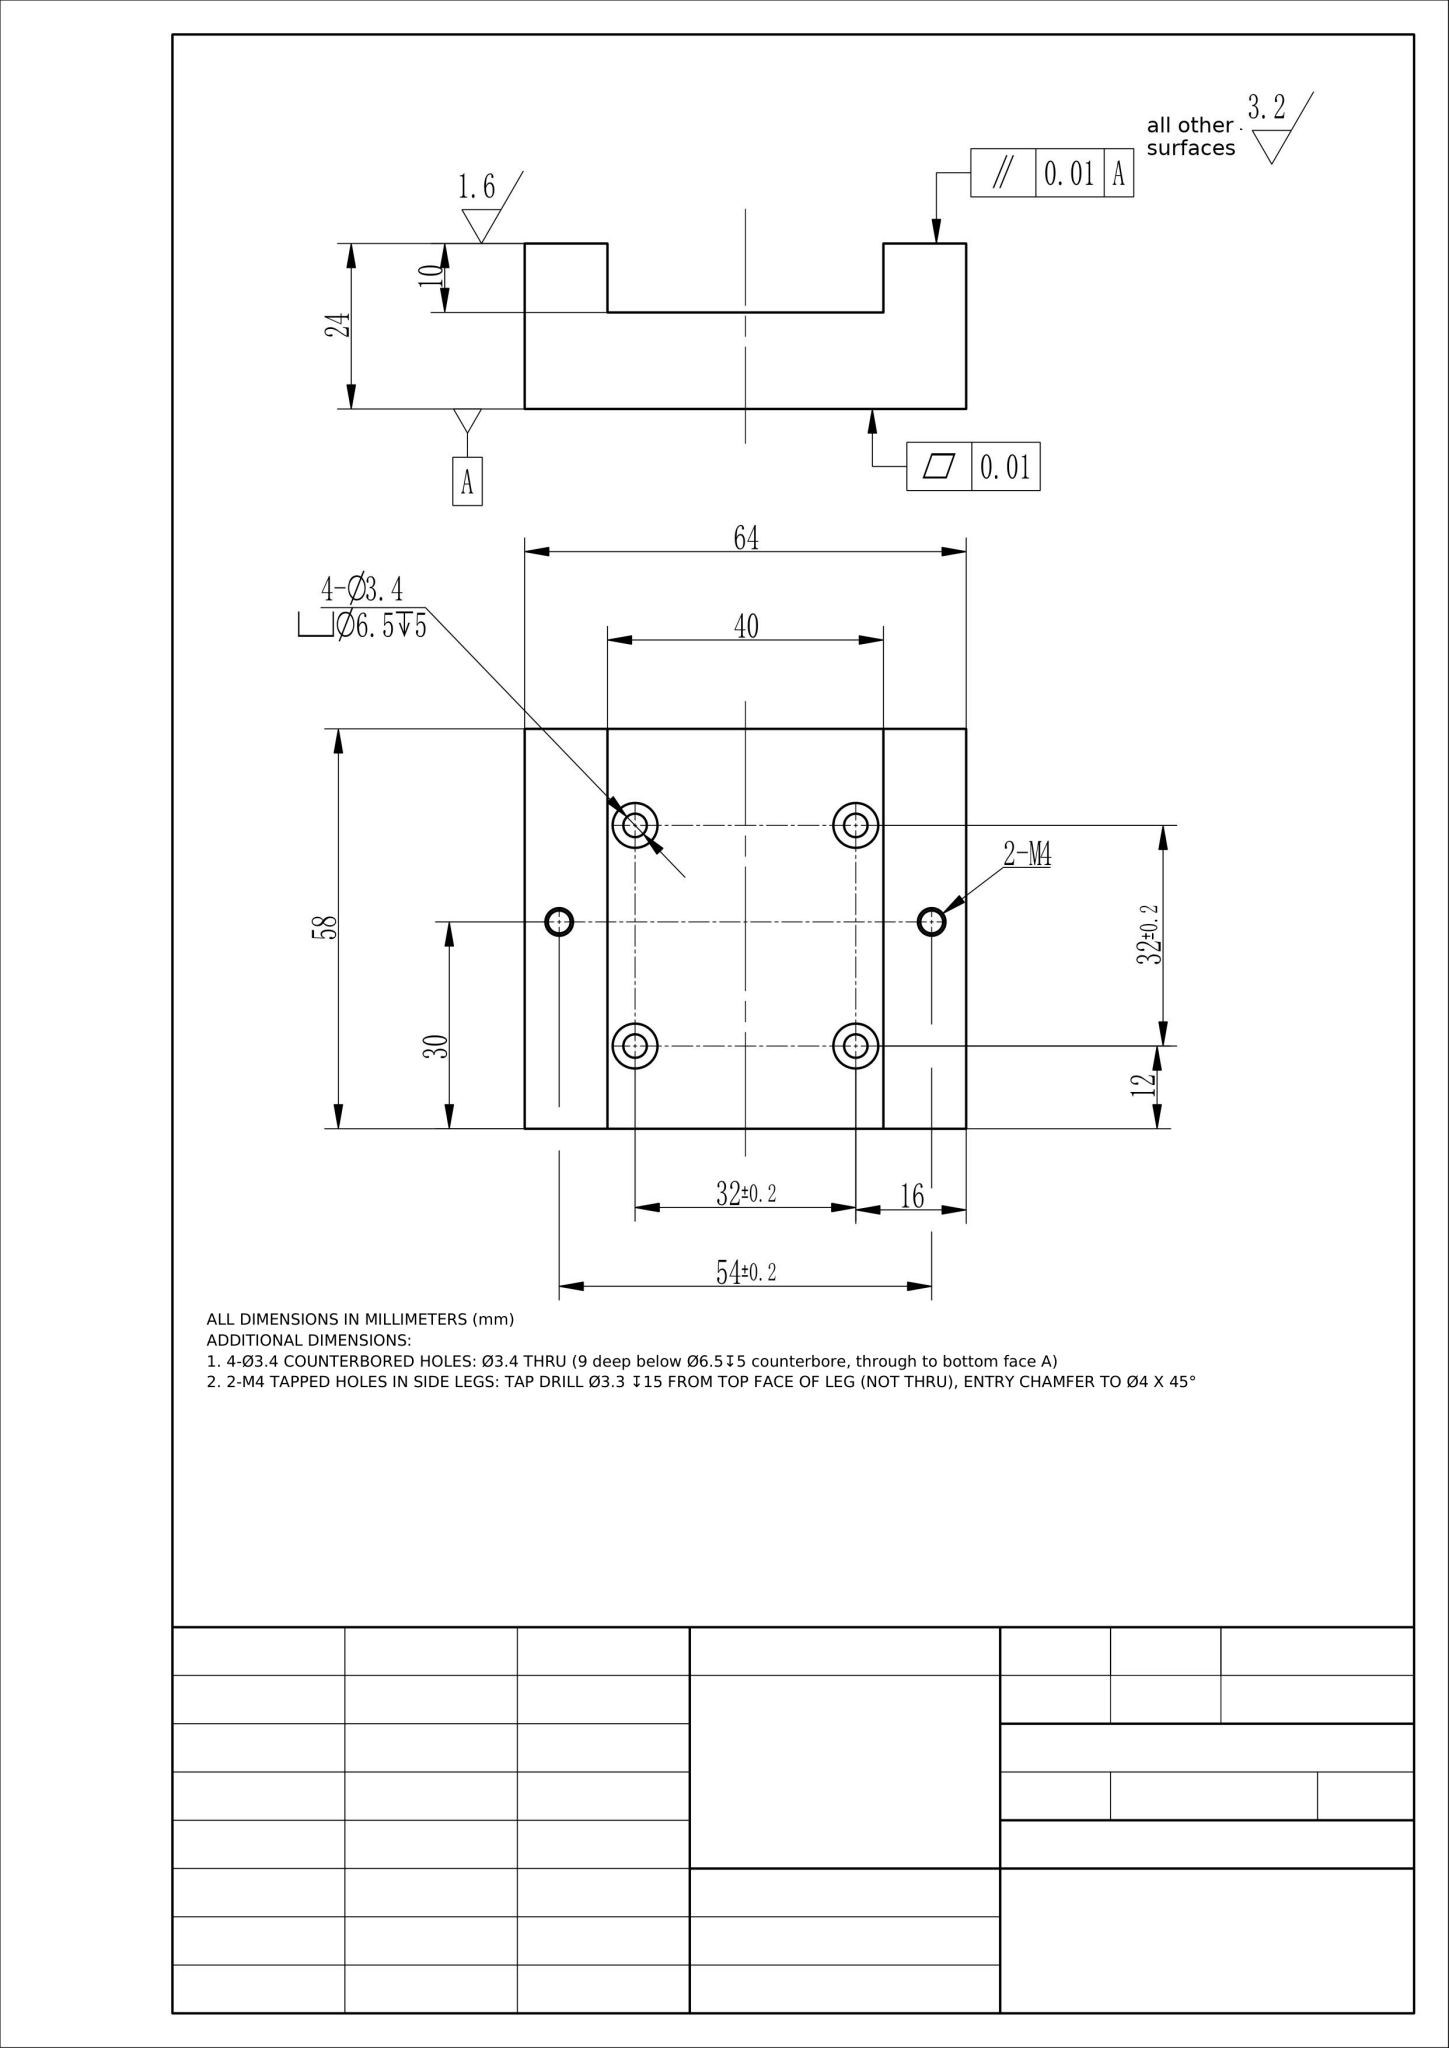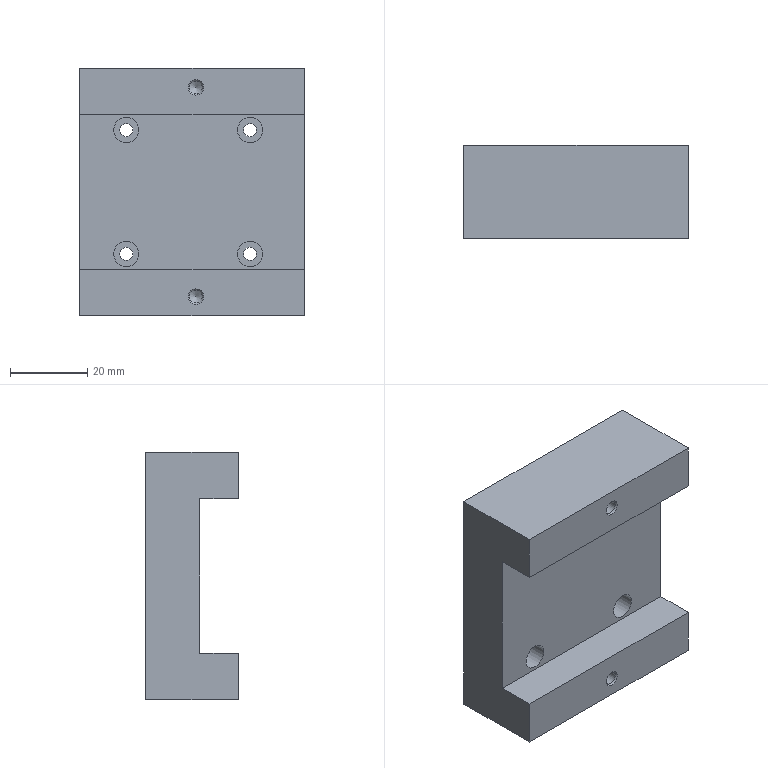Part | NX | mm | 1 solid | 28 faces | box 58 x 24 x 64 mm | volume 64634 mm3 | plane 14 | cylinder 10 | cone 4 | commonest cylinder face diameters 3.4 x4 6.5 x4 3.3 x2
STEP:
#1=CARTESIAN_POINT('',(0.,0.,0.));
#2=DIRECTION('',(0.,0.,1.));
#3=DIRECTION('',(1.,0.,0.));
#4=AXIS2_PLACEMENT_3D('',#1,#2,#3);
#5=(LENGTH_UNIT()NAMED_UNIT(*)SI_UNIT(.MILLI.,.METRE.));
#6=UNCERTAINTY_MEASURE_WITH_UNIT(LENGTH_MEASURE(0.00002),#5,'','');
#7=(NAMED_UNIT(*)PLANE_ANGLE_UNIT()SI_UNIT($,.RADIAN.));
#8=PLANE_ANGLE_MEASURE_WITH_UNIT(PLANE_ANGLE_MEASURE(0.01745),#7);
#9=DIMENSIONAL_EXPONENTS(0.,0.,0.,0.,0.,0.,0.);
#10=(CONVERSION_BASED_UNIT('',#8)NAMED_UNIT(#9)PLANE_ANGLE_UNIT());
#11=(NAMED_UNIT(*)SI_UNIT($,.STERADIAN.)SOLID_ANGLE_UNIT());
#12=(GEOMETRIC_REPRESENTATION_CONTEXT(3)GLOBAL_UNCERTAINTY_ASSIGNED_CONTEXT((#6))GLOBAL_UNIT_ASSIGNED_CONTEXT((#5,#10,#11))REPRESENTATION_CONTEXT('',''));
#13=SHAPE_REPRESENTATION('',(#4),#12);
#14=CARTESIAN_POINT('',(-56.,45.,156.029));
#15=VERTEX_POINT('',#14);
#16=CARTESIAN_POINT('',(-56.,55.,156.029));
#17=VERTEX_POINT('',#16);
#18=CARTESIAN_POINT('',(-56.,43.,156.029));
#19=DIRECTION('',(0.,1.,0.));
#20=VECTOR('',#19,1.);
#21=LINE('',#18,#20);
#22=EDGE_CURVE('',#15,#17,#21,.T.);
#23=ORIENTED_EDGE('',*,*,#22,.F.);
#24=CARTESIAN_POINT('',(-56.,45.,144.029));
#25=VERTEX_POINT('',#24);
#26=CARTESIAN_POINT('',(-56.,45.,154.029));
#27=DIRECTION('',(-0.,0.,1.));
#28=VECTOR('',#27,1.);
#29=LINE('',#26,#28);
#30=EDGE_CURVE('',#25,#15,#29,.T.);
#31=ORIENTED_EDGE('',*,*,#30,.F.);
#32=CARTESIAN_POINT('',(-56.,69.,144.029));
#33=VERTEX_POINT('',#32);
#34=CARTESIAN_POINT('',(-56.,45.,144.029));
#35=DIRECTION('',(0.,1.,0.));
#36=VECTOR('',#35,1.);
#37=LINE('',#34,#36);
#38=EDGE_CURVE('',#25,#33,#37,.T.);
#39=ORIENTED_EDGE('',*,*,#38,.T.);
#40=CARTESIAN_POINT('',(-56.,69.,208.029));
#41=VERTEX_POINT('',#40);
#42=CARTESIAN_POINT('',(-56.,69.,154.029));
#43=DIRECTION('',(-0.,0.,1.));
#44=VECTOR('',#43,1.);
#45=LINE('',#42,#44);
#46=EDGE_CURVE('',#33,#41,#45,.T.);
#47=ORIENTED_EDGE('',*,*,#46,.T.);
#48=CARTESIAN_POINT('',(-56.,45.,208.029));
#49=VERTEX_POINT('',#48);
#50=CARTESIAN_POINT('',(-56.,45.,208.029));
#51=DIRECTION('',(0.,1.,0.));
#52=VECTOR('',#51,1.);
#53=LINE('',#50,#52);
#54=EDGE_CURVE('',#49,#41,#53,.T.);
#55=ORIENTED_EDGE('',*,*,#54,.F.);
#56=CARTESIAN_POINT('',(-56.,45.,196.029));
#57=VERTEX_POINT('',#56);
#58=CARTESIAN_POINT('',(-56.,45.,154.029));
#59=DIRECTION('',(-0.,0.,1.));
#60=VECTOR('',#59,1.);
#61=LINE('',#58,#60);
#62=EDGE_CURVE('',#57,#49,#61,.T.);
#63=ORIENTED_EDGE('',*,*,#62,.F.);
#64=CARTESIAN_POINT('',(-56.,55.,196.029));
#65=VERTEX_POINT('',#64);
#66=CARTESIAN_POINT('',(-56.,55.,196.029));
#67=DIRECTION('',(0.,-1.,0.));
#68=VECTOR('',#67,1.);
#69=LINE('',#66,#68);
#70=EDGE_CURVE('',#65,#57,#69,.T.);
#71=ORIENTED_EDGE('',*,*,#70,.F.);
#72=CARTESIAN_POINT('',(-56.,55.,156.029));
#73=DIRECTION('',(0.,-0.,1.));
#74=VECTOR('',#73,1.);
#75=LINE('',#72,#74);
#76=EDGE_CURVE('',#17,#65,#75,.T.);
#77=ORIENTED_EDGE('',*,*,#76,.F.);
#78=EDGE_LOOP('',(#23,#31,#39,#47,#55,#63,#71,#77));
#79=FACE_OUTER_BOUND('',#78,.T.);
#80=CARTESIAN_POINT('',(-56.,45.,154.029));
#81=DIRECTION('',(-1.,0.,-0.));
#82=DIRECTION('',(-0.,0.,1.));
#83=AXIS2_PLACEMENT_3D('',#80,#81,#82);
#84=PLANE('',#83);
#85=ADVANCED_FACE('',(#79),#84,.F.);
#86=CARTESIAN_POINT('',(-114.,45.,156.029));
#87=VERTEX_POINT('',#86);
#88=CARTESIAN_POINT('',(0.,45.,156.029));
#89=DIRECTION('',(1.,0.,0.));
#90=VECTOR('',#89,1.);
#91=LINE('',#88,#90);
#92=EDGE_CURVE('',#87,#15,#91,.T.);
#93=ORIENTED_EDGE('',*,*,#92,.F.);
#94=CARTESIAN_POINT('',(-114.,45.,144.029));
#95=VERTEX_POINT('',#94);
#96=CARTESIAN_POINT('',(-114.,45.,198.029));
#97=DIRECTION('',(0.,0.,-1.));
#98=VECTOR('',#97,1.);
#99=LINE('',#96,#98);
#100=EDGE_CURVE('',#87,#95,#99,.T.);
#101=ORIENTED_EDGE('',*,*,#100,.T.);
#102=CARTESIAN_POINT('',(-111.,45.,144.029));
#103=DIRECTION('',(1.,0.,0.));
#104=VECTOR('',#103,1.);
#105=LINE('',#102,#104);
#106=EDGE_CURVE('',#95,#25,#105,.T.);
#107=ORIENTED_EDGE('',*,*,#106,.T.);
#108=ORIENTED_EDGE('',*,*,#30,.T.);
#109=EDGE_LOOP('',(#93,#101,#107,#108));
#110=FACE_BOUND('',#109,.T.);
#111=CARTESIAN_POINT('',(-84.,45.,147.029));
#112=VERTEX_POINT('',#111);
#113=CARTESIAN_POINT('',(-84.,45.,149.029));
#114=DIRECTION('',(0.,1.,0.));
#115=DIRECTION('',(0.,0.,-1.));
#116=AXIS2_PLACEMENT_3D('',#113,#114,#115);
#117=CIRCLE('',#116,2.);
#118=EDGE_CURVE('',#112,#112,#117,.T.);
#119=ORIENTED_EDGE('',*,*,#118,.T.);
#120=EDGE_LOOP('',(#119));
#121=FACE_BOUND('',#120,.T.);
#122=CARTESIAN_POINT('',(0.,45.,0.));
#123=DIRECTION('',(0.,-1.,0.));
#124=DIRECTION('',(0.,0.,-1.));
#125=AXIS2_PLACEMENT_3D('',#122,#123,#124);
#126=PLANE('',#125);
#127=ADVANCED_FACE('',(#110,#121),#126,.T.);
#128=ORIENTED_EDGE('',*,*,#100,.F.);
#129=CARTESIAN_POINT('',(-114.,55.,156.029));
#130=VERTEX_POINT('',#129);
#131=CARTESIAN_POINT('',(-114.,45.,156.029));
#132=DIRECTION('',(0.,1.,0.));
#133=VECTOR('',#132,1.);
#134=LINE('',#131,#133);
#135=EDGE_CURVE('',#87,#130,#134,.T.);
#136=ORIENTED_EDGE('',*,*,#135,.T.);
#137=CARTESIAN_POINT('',(-114.,55.,196.029));
#138=VERTEX_POINT('',#137);
#139=CARTESIAN_POINT('',(-114.,55.,198.029));
#140=DIRECTION('',(-0.,-0.,1.));
#141=VECTOR('',#140,1.);
#142=LINE('',#139,#141);
#143=EDGE_CURVE('',#130,#138,#142,.T.);
#144=ORIENTED_EDGE('',*,*,#143,.T.);
#145=CARTESIAN_POINT('',(-114.,45.,196.029));
#146=VERTEX_POINT('',#145);
#147=CARTESIAN_POINT('',(-114.,45.,196.029));
#148=DIRECTION('',(0.,-1.,0.));
#149=VECTOR('',#148,1.);
#150=LINE('',#147,#149);
#151=EDGE_CURVE('',#138,#146,#150,.T.);
#152=ORIENTED_EDGE('',*,*,#151,.T.);
#153=CARTESIAN_POINT('',(-114.,45.,208.029));
#154=VERTEX_POINT('',#153);
#155=CARTESIAN_POINT('',(-114.,45.,198.029));
#156=DIRECTION('',(0.,0.,-1.));
#157=VECTOR('',#156,1.);
#158=LINE('',#155,#157);
#159=EDGE_CURVE('',#154,#146,#158,.T.);
#160=ORIENTED_EDGE('',*,*,#159,.F.);
#161=CARTESIAN_POINT('',(-114.,69.,208.029));
#162=VERTEX_POINT('',#161);
#163=CARTESIAN_POINT('',(-114.,45.,208.029));
#164=DIRECTION('',(0.,1.,0.));
#165=VECTOR('',#164,1.);
#166=LINE('',#163,#165);
#167=EDGE_CURVE('',#154,#162,#166,.T.);
#168=ORIENTED_EDGE('',*,*,#167,.T.);
#169=CARTESIAN_POINT('',(-114.,69.,144.029));
#170=VERTEX_POINT('',#169);
#171=CARTESIAN_POINT('',(-114.,69.,198.029));
#172=DIRECTION('',(0.,0.,-1.));
#173=VECTOR('',#172,1.);
#174=LINE('',#171,#173);
#175=EDGE_CURVE('',#162,#170,#174,.T.);
#176=ORIENTED_EDGE('',*,*,#175,.T.);
#177=CARTESIAN_POINT('',(-114.,45.,144.029));
#178=DIRECTION('',(0.,1.,0.));
#179=VECTOR('',#178,1.);
#180=LINE('',#177,#179);
#181=EDGE_CURVE('',#95,#170,#180,.T.);
#182=ORIENTED_EDGE('',*,*,#181,.F.);
#183=EDGE_LOOP('',(#128,#136,#144,#152,#160,#168,#176,#182));
#184=FACE_OUTER_BOUND('',#183,.T.);
#185=CARTESIAN_POINT('',(-114.,45.,198.029));
#186=DIRECTION('',(1.,0.,0.));
#187=DIRECTION('',(0.,0.,-1.));
#188=AXIS2_PLACEMENT_3D('',#185,#186,#187);
#189=PLANE('',#188);
#190=ADVANCED_FACE('',(#184),#189,.F.);
#191=CARTESIAN_POINT('',(-111.,69.,144.029));
#192=DIRECTION('',(1.,0.,0.));
#193=VECTOR('',#192,1.);
#194=LINE('',#191,#193);
#195=EDGE_CURVE('',#170,#33,#194,.T.);
#196=ORIENTED_EDGE('',*,*,#195,.T.);
#197=ORIENTED_EDGE('',*,*,#38,.F.);
#198=ORIENTED_EDGE('',*,*,#106,.F.);
#199=ORIENTED_EDGE('',*,*,#181,.T.);
#200=EDGE_LOOP('',(#196,#197,#198,#199));
#201=FACE_OUTER_BOUND('',#200,.T.);
#202=CARTESIAN_POINT('',(-111.,45.,144.029));
#203=DIRECTION('',(0.,0.,1.));
#204=DIRECTION('',(1.,0.,0.));
#205=AXIS2_PLACEMENT_3D('',#202,#203,#204);
#206=PLANE('',#205);
#207=ADVANCED_FACE('',(#201),#206,.F.);
#208=CARTESIAN_POINT('',(-61.,69.,208.029));
#209=DIRECTION('',(-1.,0.,0.));
#210=VECTOR('',#209,1.);
#211=LINE('',#208,#210);
#212=EDGE_CURVE('',#41,#162,#211,.T.);
#213=ORIENTED_EDGE('',*,*,#212,.T.);
#214=ORIENTED_EDGE('',*,*,#167,.F.);
#215=CARTESIAN_POINT('',(-61.,45.,208.029));
#216=DIRECTION('',(-1.,0.,0.));
#217=VECTOR('',#216,1.);
#218=LINE('',#215,#217);
#219=EDGE_CURVE('',#49,#154,#218,.T.);
#220=ORIENTED_EDGE('',*,*,#219,.F.);
#221=ORIENTED_EDGE('',*,*,#54,.T.);
#222=EDGE_LOOP('',(#213,#214,#220,#221));
#223=FACE_OUTER_BOUND('',#222,.T.);
#224=CARTESIAN_POINT('',(-61.,45.,208.029));
#225=DIRECTION('',(0.,0.,-1.));
#226=DIRECTION('',(-1.,0.,0.));
#227=AXIS2_PLACEMENT_3D('',#224,#225,#226);
#228=PLANE('',#227);
#229=ADVANCED_FACE('',(#223),#228,.F.);
#230=CARTESIAN_POINT('',(0.,45.,196.029));
#231=DIRECTION('',(-1.,0.,0.));
#232=VECTOR('',#231,1.);
#233=LINE('',#230,#232);
#234=EDGE_CURVE('',#57,#146,#233,.T.);
#235=ORIENTED_EDGE('',*,*,#234,.F.);
#236=ORIENTED_EDGE('',*,*,#62,.T.);
#237=ORIENTED_EDGE('',*,*,#219,.T.);
#238=ORIENTED_EDGE('',*,*,#159,.T.);
#239=EDGE_LOOP('',(#235,#236,#237,#238));
#240=FACE_BOUND('',#239,.T.);
#241=CARTESIAN_POINT('',(-84.,45.,201.029));
#242=VERTEX_POINT('',#241);
#243=CARTESIAN_POINT('',(-84.,45.,203.029));
#244=DIRECTION('',(0.,1.,0.));
#245=DIRECTION('',(0.,0.,-1.));
#246=AXIS2_PLACEMENT_3D('',#243,#244,#245);
#247=CIRCLE('',#246,2.);
#248=EDGE_CURVE('',#242,#242,#247,.T.);
#249=ORIENTED_EDGE('',*,*,#248,.T.);
#250=EDGE_LOOP('',(#249));
#251=FACE_BOUND('',#250,.T.);
#252=CARTESIAN_POINT('',(0.,45.,0.));
#253=DIRECTION('',(0.,-1.,0.));
#254=DIRECTION('',(0.,0.,-1.));
#255=AXIS2_PLACEMENT_3D('',#252,#253,#254);
#256=PLANE('',#255);
#257=ADVANCED_FACE('',(#240,#251),#256,.T.);
#258=CARTESIAN_POINT('',(-70.,69.,158.329));
#259=VERTEX_POINT('',#258);
#260=CARTESIAN_POINT('',(-70.,69.,160.029));
#261=DIRECTION('',(0.,-1.,0.));
#262=DIRECTION('',(0.,0.,-1.));
#263=AXIS2_PLACEMENT_3D('',#260,#261,#262);
#264=CIRCLE('',#263,1.7);
#265=EDGE_CURVE('',#259,#259,#264,.T.);
#266=ORIENTED_EDGE('',*,*,#265,.T.);
#267=EDGE_LOOP('',(#266));
#268=FACE_BOUND('',#267,.T.);
#269=CARTESIAN_POINT('',(-102.,69.,158.329));
#270=VERTEX_POINT('',#269);
#271=CARTESIAN_POINT('',(-102.,69.,160.029));
#272=DIRECTION('',(0.,-1.,0.));
#273=DIRECTION('',(0.,0.,-1.));
#274=AXIS2_PLACEMENT_3D('',#271,#272,#273);
#275=CIRCLE('',#274,1.7);
#276=EDGE_CURVE('',#270,#270,#275,.T.);
#277=ORIENTED_EDGE('',*,*,#276,.T.);
#278=EDGE_LOOP('',(#277));
#279=FACE_BOUND('',#278,.T.);
#280=CARTESIAN_POINT('',(-70.,69.,190.329));
#281=VERTEX_POINT('',#280);
#282=CARTESIAN_POINT('',(-70.,69.,192.029));
#283=DIRECTION('',(0.,-1.,0.));
#284=DIRECTION('',(0.,0.,-1.));
#285=AXIS2_PLACEMENT_3D('',#282,#283,#284);
#286=CIRCLE('',#285,1.7);
#287=EDGE_CURVE('',#281,#281,#286,.T.);
#288=ORIENTED_EDGE('',*,*,#287,.T.);
#289=EDGE_LOOP('',(#288));
#290=FACE_BOUND('',#289,.T.);
#291=CARTESIAN_POINT('',(-102.,69.,190.329));
#292=VERTEX_POINT('',#291);
#293=CARTESIAN_POINT('',(-102.,69.,192.029));
#294=DIRECTION('',(0.,-1.,0.));
#295=DIRECTION('',(0.,0.,-1.));
#296=AXIS2_PLACEMENT_3D('',#293,#294,#295);
#297=CIRCLE('',#296,1.7);
#298=EDGE_CURVE('',#292,#292,#297,.T.);
#299=ORIENTED_EDGE('',*,*,#298,.T.);
#300=EDGE_LOOP('',(#299));
#301=FACE_BOUND('',#300,.T.);
#302=ORIENTED_EDGE('',*,*,#175,.F.);
#303=ORIENTED_EDGE('',*,*,#212,.F.);
#304=ORIENTED_EDGE('',*,*,#46,.F.);
#305=ORIENTED_EDGE('',*,*,#195,.F.);
#306=EDGE_LOOP('',(#302,#303,#304,#305));
#307=FACE_BOUND('',#306,.T.);
#308=CARTESIAN_POINT('',(0.,69.,0.));
#309=DIRECTION('',(0.,-1.,0.));
#310=DIRECTION('',(0.,0.,-1.));
#311=AXIS2_PLACEMENT_3D('',#308,#309,#310);
#312=PLANE('',#311);
#313=ADVANCED_FACE('',(#268,#279,#290,#301,#307),#312,.F.);
#314=CARTESIAN_POINT('',(-102.,60.,193.729));
#315=VERTEX_POINT('',#314);
#316=CARTESIAN_POINT('',(-102.,60.,192.029));
#317=DIRECTION('',(0.,-1.,0.));
#318=DIRECTION('',(0.,0.,1.));
#319=AXIS2_PLACEMENT_3D('',#316,#317,#318);
#320=CIRCLE('',#319,1.7);
#321=EDGE_CURVE('',#315,#315,#320,.T.);
#322=ORIENTED_EDGE('',*,*,#321,.T.);
#323=EDGE_LOOP('',(#322));
#324=FACE_BOUND('',#323,.T.);
#325=ORIENTED_EDGE('',*,*,#298,.F.);
#326=EDGE_LOOP('',(#325));
#327=FACE_BOUND('',#326,.T.);
#328=CARTESIAN_POINT('',(-102.,95.,192.029));
#329=DIRECTION('',(0.,1.,0.));
#330=DIRECTION('',(0.,0.,1.));
#331=AXIS2_PLACEMENT_3D('',#328,#329,#330);
#332=CYLINDRICAL_SURFACE('',#331,1.7);
#333=ADVANCED_FACE('',(#324,#327),#332,.F.);
#334=ORIENTED_EDGE('',*,*,#321,.F.);
#335=EDGE_LOOP('',(#334));
#336=FACE_BOUND('',#335,.T.);
#337=CARTESIAN_POINT('',(-102.,60.,195.279));
#338=VERTEX_POINT('',#337);
#339=CARTESIAN_POINT('',(-102.,60.,192.029));
#340=DIRECTION('',(0.,-1.,0.));
#341=DIRECTION('',(0.,0.,1.));
#342=AXIS2_PLACEMENT_3D('',#339,#340,#341);
#343=CIRCLE('',#342,3.25);
#344=EDGE_CURVE('',#338,#338,#343,.T.);
#345=ORIENTED_EDGE('',*,*,#344,.T.);
#346=EDGE_LOOP('',(#345));
#347=FACE_BOUND('',#346,.T.);
#348=CARTESIAN_POINT('',(-102.,60.,192.029));
#349=DIRECTION('',(0.,1.,0.));
#350=DIRECTION('',(0.,0.,1.));
#351=AXIS2_PLACEMENT_3D('',#348,#349,#350);
#352=PLANE('',#351);
#353=ADVANCED_FACE('',(#336,#347),#352,.F.);
#354=CARTESIAN_POINT('',(-102.,55.,195.279));
#355=VERTEX_POINT('',#354);
#356=CARTESIAN_POINT('',(-102.,55.,192.029));
#357=DIRECTION('',(0.,-1.,-0.));
#358=DIRECTION('',(0.,0.,1.));
#359=AXIS2_PLACEMENT_3D('',#356,#357,#358);
#360=CIRCLE('',#359,3.25);
#361=EDGE_CURVE('',#355,#355,#360,.T.);
#362=ORIENTED_EDGE('',*,*,#361,.T.);
#363=EDGE_LOOP('',(#362));
#364=FACE_BOUND('',#363,.T.);
#365=ORIENTED_EDGE('',*,*,#344,.F.);
#366=EDGE_LOOP('',(#365));
#367=FACE_BOUND('',#366,.T.);
#368=CARTESIAN_POINT('',(-102.,45.,192.029));
#369=DIRECTION('',(0.,1.,0.));
#370=DIRECTION('',(0.,0.,1.));
#371=AXIS2_PLACEMENT_3D('',#368,#369,#370);
#372=CYLINDRICAL_SURFACE('',#371,3.25);
#373=ADVANCED_FACE('',(#364,#367),#372,.F.);
#374=CARTESIAN_POINT('',(-70.,60.,193.729));
#375=VERTEX_POINT('',#374);
#376=CARTESIAN_POINT('',(-70.,60.,192.029));
#377=DIRECTION('',(0.,-1.,0.));
#378=DIRECTION('',(0.,0.,1.));
#379=AXIS2_PLACEMENT_3D('',#376,#377,#378);
#380=CIRCLE('',#379,1.7);
#381=EDGE_CURVE('',#375,#375,#380,.T.);
#382=ORIENTED_EDGE('',*,*,#381,.T.);
#383=EDGE_LOOP('',(#382));
#384=FACE_BOUND('',#383,.T.);
#385=ORIENTED_EDGE('',*,*,#287,.F.);
#386=EDGE_LOOP('',(#385));
#387=FACE_BOUND('',#386,.T.);
#388=CARTESIAN_POINT('',(-70.,95.,192.029));
#389=DIRECTION('',(0.,1.,0.));
#390=DIRECTION('',(0.,0.,1.));
#391=AXIS2_PLACEMENT_3D('',#388,#389,#390);
#392=CYLINDRICAL_SURFACE('',#391,1.7);
#393=ADVANCED_FACE('',(#384,#387),#392,.F.);
#394=ORIENTED_EDGE('',*,*,#381,.F.);
#395=EDGE_LOOP('',(#394));
#396=FACE_BOUND('',#395,.T.);
#397=CARTESIAN_POINT('',(-70.,60.,195.279));
#398=VERTEX_POINT('',#397);
#399=CARTESIAN_POINT('',(-70.,60.,192.029));
#400=DIRECTION('',(0.,-1.,0.));
#401=DIRECTION('',(0.,0.,1.));
#402=AXIS2_PLACEMENT_3D('',#399,#400,#401);
#403=CIRCLE('',#402,3.25);
#404=EDGE_CURVE('',#398,#398,#403,.T.);
#405=ORIENTED_EDGE('',*,*,#404,.T.);
#406=EDGE_LOOP('',(#405));
#407=FACE_BOUND('',#406,.T.);
#408=CARTESIAN_POINT('',(-70.,60.,192.029));
#409=DIRECTION('',(0.,1.,0.));
#410=DIRECTION('',(0.,0.,1.));
#411=AXIS2_PLACEMENT_3D('',#408,#409,#410);
#412=PLANE('',#411);
#413=ADVANCED_FACE('',(#396,#407),#412,.F.);
#414=CARTESIAN_POINT('',(-70.,55.,195.279));
#415=VERTEX_POINT('',#414);
#416=CARTESIAN_POINT('',(-70.,55.,192.029));
#417=DIRECTION('',(0.,-1.,-0.));
#418=DIRECTION('',(0.,0.,1.));
#419=AXIS2_PLACEMENT_3D('',#416,#417,#418);
#420=CIRCLE('',#419,3.25);
#421=EDGE_CURVE('',#415,#415,#420,.T.);
#422=ORIENTED_EDGE('',*,*,#421,.T.);
#423=EDGE_LOOP('',(#422));
#424=FACE_BOUND('',#423,.T.);
#425=ORIENTED_EDGE('',*,*,#404,.F.);
#426=EDGE_LOOP('',(#425));
#427=FACE_BOUND('',#426,.T.);
#428=CARTESIAN_POINT('',(-70.,45.,192.029));
#429=DIRECTION('',(0.,1.,0.));
#430=DIRECTION('',(0.,0.,1.));
#431=AXIS2_PLACEMENT_3D('',#428,#429,#430);
#432=CYLINDRICAL_SURFACE('',#431,3.25);
#433=ADVANCED_FACE('',(#424,#427),#432,.F.);
#434=CARTESIAN_POINT('',(-102.,60.,161.729));
#435=VERTEX_POINT('',#434);
#436=CARTESIAN_POINT('',(-102.,60.,160.029));
#437=DIRECTION('',(0.,-1.,0.));
#438=DIRECTION('',(0.,0.,1.));
#439=AXIS2_PLACEMENT_3D('',#436,#437,#438);
#440=CIRCLE('',#439,1.7);
#441=EDGE_CURVE('',#435,#435,#440,.T.);
#442=ORIENTED_EDGE('',*,*,#441,.T.);
#443=EDGE_LOOP('',(#442));
#444=FACE_BOUND('',#443,.T.);
#445=ORIENTED_EDGE('',*,*,#276,.F.);
#446=EDGE_LOOP('',(#445));
#447=FACE_BOUND('',#446,.T.);
#448=CARTESIAN_POINT('',(-102.,95.,160.029));
#449=DIRECTION('',(0.,1.,0.));
#450=DIRECTION('',(0.,0.,1.));
#451=AXIS2_PLACEMENT_3D('',#448,#449,#450);
#452=CYLINDRICAL_SURFACE('',#451,1.7);
#453=ADVANCED_FACE('',(#444,#447),#452,.F.);
#454=ORIENTED_EDGE('',*,*,#441,.F.);
#455=EDGE_LOOP('',(#454));
#456=FACE_BOUND('',#455,.T.);
#457=CARTESIAN_POINT('',(-102.,60.,163.279));
#458=VERTEX_POINT('',#457);
#459=CARTESIAN_POINT('',(-102.,60.,160.029));
#460=DIRECTION('',(0.,-1.,0.));
#461=DIRECTION('',(0.,0.,1.));
#462=AXIS2_PLACEMENT_3D('',#459,#460,#461);
#463=CIRCLE('',#462,3.25);
#464=EDGE_CURVE('',#458,#458,#463,.T.);
#465=ORIENTED_EDGE('',*,*,#464,.T.);
#466=EDGE_LOOP('',(#465));
#467=FACE_BOUND('',#466,.T.);
#468=CARTESIAN_POINT('',(-102.,60.,160.029));
#469=DIRECTION('',(0.,1.,0.));
#470=DIRECTION('',(0.,0.,1.));
#471=AXIS2_PLACEMENT_3D('',#468,#469,#470);
#472=PLANE('',#471);
#473=ADVANCED_FACE('',(#456,#467),#472,.F.);
#474=CARTESIAN_POINT('',(-102.,55.,163.279));
#475=VERTEX_POINT('',#474);
#476=CARTESIAN_POINT('',(-102.,55.,160.029));
#477=DIRECTION('',(0.,-1.,-0.));
#478=DIRECTION('',(0.,0.,1.));
#479=AXIS2_PLACEMENT_3D('',#476,#477,#478);
#480=CIRCLE('',#479,3.25);
#481=EDGE_CURVE('',#475,#475,#480,.T.);
#482=ORIENTED_EDGE('',*,*,#481,.T.);
#483=EDGE_LOOP('',(#482));
#484=FACE_BOUND('',#483,.T.);
#485=ORIENTED_EDGE('',*,*,#464,.F.);
#486=EDGE_LOOP('',(#485));
#487=FACE_BOUND('',#486,.T.);
#488=CARTESIAN_POINT('',(-102.,45.,160.029));
#489=DIRECTION('',(0.,1.,0.));
#490=DIRECTION('',(0.,0.,1.));
#491=AXIS2_PLACEMENT_3D('',#488,#489,#490);
#492=CYLINDRICAL_SURFACE('',#491,3.25);
#493=ADVANCED_FACE('',(#484,#487),#492,.F.);
#494=CARTESIAN_POINT('',(-70.,60.,161.729));
#495=VERTEX_POINT('',#494);
#496=CARTESIAN_POINT('',(-70.,60.,160.029));
#497=DIRECTION('',(0.,-1.,0.));
#498=DIRECTION('',(0.,0.,1.));
#499=AXIS2_PLACEMENT_3D('',#496,#497,#498);
#500=CIRCLE('',#499,1.7);
#501=EDGE_CURVE('',#495,#495,#500,.T.);
#502=ORIENTED_EDGE('',*,*,#501,.T.);
#503=EDGE_LOOP('',(#502));
#504=FACE_BOUND('',#503,.T.);
#505=ORIENTED_EDGE('',*,*,#265,.F.);
#506=EDGE_LOOP('',(#505));
#507=FACE_BOUND('',#506,.T.);
#508=CARTESIAN_POINT('',(-70.,95.,160.029));
#509=DIRECTION('',(0.,1.,0.));
#510=DIRECTION('',(0.,0.,1.));
#511=AXIS2_PLACEMENT_3D('',#508,#509,#510);
#512=CYLINDRICAL_SURFACE('',#511,1.7);
#513=ADVANCED_FACE('',(#504,#507),#512,.F.);
#514=ORIENTED_EDGE('',*,*,#501,.F.);
#515=EDGE_LOOP('',(#514));
#516=FACE_BOUND('',#515,.T.);
#517=CARTESIAN_POINT('',(-70.,60.,163.279));
#518=VERTEX_POINT('',#517);
#519=CARTESIAN_POINT('',(-70.,60.,160.029));
#520=DIRECTION('',(0.,-1.,0.));
#521=DIRECTION('',(0.,0.,1.));
#522=AXIS2_PLACEMENT_3D('',#519,#520,#521);
#523=CIRCLE('',#522,3.25);
#524=EDGE_CURVE('',#518,#518,#523,.T.);
#525=ORIENTED_EDGE('',*,*,#524,.T.);
#526=EDGE_LOOP('',(#525));
#527=FACE_BOUND('',#526,.T.);
#528=CARTESIAN_POINT('',(-70.,60.,160.029));
#529=DIRECTION('',(0.,1.,0.));
#530=DIRECTION('',(0.,0.,1.));
#531=AXIS2_PLACEMENT_3D('',#528,#529,#530);
#532=PLANE('',#531);
#533=ADVANCED_FACE('',(#516,#527),#532,.F.);
#534=CARTESIAN_POINT('',(-70.,55.,163.279));
#535=VERTEX_POINT('',#534);
#536=CARTESIAN_POINT('',(-70.,55.,160.029));
#537=DIRECTION('',(0.,-1.,-0.));
#538=DIRECTION('',(0.,0.,1.));
#539=AXIS2_PLACEMENT_3D('',#536,#537,#538);
#540=CIRCLE('',#539,3.25);
#541=EDGE_CURVE('',#535,#535,#540,.T.);
#542=ORIENTED_EDGE('',*,*,#541,.T.);
#543=EDGE_LOOP('',(#542));
#544=FACE_BOUND('',#543,.T.);
#545=ORIENTED_EDGE('',*,*,#524,.F.);
#546=EDGE_LOOP('',(#545));
#547=FACE_BOUND('',#546,.T.);
#548=CARTESIAN_POINT('',(-70.,45.,160.029));
#549=DIRECTION('',(0.,1.,0.));
#550=DIRECTION('',(0.,0.,1.));
#551=AXIS2_PLACEMENT_3D('',#548,#549,#550);
#552=CYLINDRICAL_SURFACE('',#551,3.25);
#553=ADVANCED_FACE('',(#544,#547),#552,.F.);
#554=CARTESIAN_POINT('',(-84.,60.,150.679));
#555=VERTEX_POINT('',#554);
#556=CARTESIAN_POINT('',(-84.,60.,149.029));
#557=DIRECTION('',(0.,-1.,0.));
#558=DIRECTION('',(0.,0.,1.));
#559=AXIS2_PLACEMENT_3D('',#556,#557,#558);
#560=CIRCLE('',#559,1.65);
#561=EDGE_CURVE('',#555,#555,#560,.T.);
#562=ORIENTED_EDGE('',*,*,#561,.T.);
#563=EDGE_LOOP('',(#562));
#564=FACE_BOUND('',#563,.T.);
#565=CARTESIAN_POINT('',(-84.,60.991,149.029));
#566=VERTEX_POINT('',#565);
#567=VERTEX_LOOP('',#566);
#568=FACE_BOUND('',#567,.T.);
#569=CARTESIAN_POINT('',(-84.,60.,149.029));
#570=DIRECTION('',(0.,-1.,0.));
#571=DIRECTION('',(0.,0.,-1.));
#572=AXIS2_PLACEMENT_3D('',#569,#570,#571);
#573=CONICAL_SURFACE('',#572,1.65,59.);
#574=ADVANCED_FACE('',(#564,#568),#573,.F.);
#575=CARTESIAN_POINT('',(-84.,45.35,147.379));
#576=VERTEX_POINT('',#575);
#577=CARTESIAN_POINT('',(-84.,45.35,149.029));
#578=DIRECTION('',(0.,-1.,0.));
#579=DIRECTION('',(0.,0.,-1.));
#580=AXIS2_PLACEMENT_3D('',#577,#578,#579);
#581=CIRCLE('',#580,1.65);
#582=EDGE_CURVE('',#576,#576,#581,.T.);
#583=ORIENTED_EDGE('',*,*,#582,.T.);
#584=EDGE_LOOP('',(#583));
#585=FACE_BOUND('',#584,.T.);
#586=ORIENTED_EDGE('',*,*,#561,.F.);
#587=EDGE_LOOP('',(#586));
#588=FACE_BOUND('',#587,.T.);
#589=CARTESIAN_POINT('',(-84.,45.,149.029));
#590=DIRECTION('',(0.,1.,0.));
#591=DIRECTION('',(0.,0.,1.));
#592=AXIS2_PLACEMENT_3D('',#589,#590,#591);
#593=CYLINDRICAL_SURFACE('',#592,1.65);
#594=ADVANCED_FACE('',(#585,#588),#593,.F.);
#595=ORIENTED_EDGE('',*,*,#582,.F.);
#596=EDGE_LOOP('',(#595));
#597=FACE_BOUND('',#596,.T.);
#598=ORIENTED_EDGE('',*,*,#118,.F.);
#599=EDGE_LOOP('',(#598));
#600=FACE_BOUND('',#599,.T.);
#601=CARTESIAN_POINT('',(-84.,45.,149.029));
#602=DIRECTION('',(0.,-1.,0.));
#603=DIRECTION('',(0.,0.,-1.));
#604=AXIS2_PLACEMENT_3D('',#601,#602,#603);
#605=CONICAL_SURFACE('',#604,2.,45.);
#606=ADVANCED_FACE('',(#597,#600),#605,.F.);
#607=CARTESIAN_POINT('',(-84.,60.,204.679));
#608=VERTEX_POINT('',#607);
#609=CARTESIAN_POINT('',(-84.,60.,203.029));
#610=DIRECTION('',(0.,-1.,0.));
#611=DIRECTION('',(0.,0.,1.));
#612=AXIS2_PLACEMENT_3D('',#609,#610,#611);
#613=CIRCLE('',#612,1.65);
#614=EDGE_CURVE('',#608,#608,#613,.T.);
#615=ORIENTED_EDGE('',*,*,#614,.T.);
#616=EDGE_LOOP('',(#615));
#617=FACE_BOUND('',#616,.T.);
#618=CARTESIAN_POINT('',(-84.,60.991,203.029));
#619=VERTEX_POINT('',#618);
#620=VERTEX_LOOP('',#619);
#621=FACE_BOUND('',#620,.T.);
#622=CARTESIAN_POINT('',(-84.,60.,203.029));
#623=DIRECTION('',(0.,-1.,0.));
#624=DIRECTION('',(0.,0.,-1.));
#625=AXIS2_PLACEMENT_3D('',#622,#623,#624);
#626=CONICAL_SURFACE('',#625,1.65,59.);
#627=ADVANCED_FACE('',(#617,#621),#626,.F.);
#628=CARTESIAN_POINT('',(-84.,45.35,201.379));
#629=VERTEX_POINT('',#628);
#630=CARTESIAN_POINT('',(-84.,45.35,203.029));
#631=DIRECTION('',(0.,-1.,0.));
#632=DIRECTION('',(0.,0.,-1.));
#633=AXIS2_PLACEMENT_3D('',#630,#631,#632);
#634=CIRCLE('',#633,1.65);
#635=EDGE_CURVE('',#629,#629,#634,.T.);
#636=ORIENTED_EDGE('',*,*,#635,.T.);
#637=EDGE_LOOP('',(#636));
#638=FACE_BOUND('',#637,.T.);
#639=ORIENTED_EDGE('',*,*,#614,.F.);
#640=EDGE_LOOP('',(#639));
#641=FACE_BOUND('',#640,.T.);
#642=CARTESIAN_POINT('',(-84.,45.,203.029));
#643=DIRECTION('',(0.,1.,0.));
#644=DIRECTION('',(0.,0.,1.));
#645=AXIS2_PLACEMENT_3D('',#642,#643,#644);
#646=CYLINDRICAL_SURFACE('',#645,1.65);
#647=ADVANCED_FACE('',(#638,#641),#646,.F.);
#648=ORIENTED_EDGE('',*,*,#635,.F.);
#649=EDGE_LOOP('',(#648));
#650=FACE_BOUND('',#649,.T.);
#651=ORIENTED_EDGE('',*,*,#248,.F.);
#652=EDGE_LOOP('',(#651));
#653=FACE_BOUND('',#652,.T.);
#654=CARTESIAN_POINT('',(-84.,45.,203.029));
#655=DIRECTION('',(0.,-1.,0.));
#656=DIRECTION('',(0.,0.,-1.));
#657=AXIS2_PLACEMENT_3D('',#654,#655,#656);
#658=CONICAL_SURFACE('',#657,2.,45.);
#659=ADVANCED_FACE('',(#650,#653),#658,.F.);
#660=ORIENTED_EDGE('',*,*,#92,.T.);
#661=ORIENTED_EDGE('',*,*,#22,.T.);
#662=CARTESIAN_POINT('',(-147.,55.,156.029));
#663=DIRECTION('',(-1.,0.,0.));
#664=VECTOR('',#663,1.);
#665=LINE('',#662,#664);
#666=EDGE_CURVE('',#17,#130,#665,.T.);
#667=ORIENTED_EDGE('',*,*,#666,.T.);
#668=ORIENTED_EDGE('',*,*,#135,.F.);
#669=EDGE_LOOP('',(#660,#661,#667,#668));
#670=FACE_OUTER_BOUND('',#669,.T.);
#671=CARTESIAN_POINT('',(-147.,43.,156.029));
#672=DIRECTION('',(0.,0.,-1.));
#673=DIRECTION('',(-1.,0.,0.));
#674=AXIS2_PLACEMENT_3D('',#671,#672,#673);
#675=PLANE('',#674);
#676=ADVANCED_FACE('',(#670),#675,.F.);
#677=CARTESIAN_POINT('',(-147.,55.,196.029));
#678=DIRECTION('',(-1.,0.,0.));
#679=VECTOR('',#678,1.);
#680=LINE('',#677,#679);
#681=EDGE_CURVE('',#65,#138,#680,.T.);
#682=ORIENTED_EDGE('',*,*,#681,.F.);
#683=ORIENTED_EDGE('',*,*,#70,.T.);
#684=ORIENTED_EDGE('',*,*,#234,.T.);
#685=ORIENTED_EDGE('',*,*,#151,.F.);
#686=EDGE_LOOP('',(#682,#683,#684,#685));
#687=FACE_OUTER_BOUND('',#686,.T.);
#688=CARTESIAN_POINT('',(-147.,55.,196.029));
#689=DIRECTION('',(0.,0.,1.));
#690=DIRECTION('',(1.,0.,0.));
#691=AXIS2_PLACEMENT_3D('',#688,#689,#690);
#692=PLANE('',#691);
#693=ADVANCED_FACE('',(#687),#692,.F.);
#694=ORIENTED_EDGE('',*,*,#421,.F.);
#695=EDGE_LOOP('',(#694));
#696=FACE_BOUND('',#695,.T.);
#697=ORIENTED_EDGE('',*,*,#541,.F.);
#698=EDGE_LOOP('',(#697));
#699=FACE_BOUND('',#698,.T.);
#700=ORIENTED_EDGE('',*,*,#481,.F.);
#701=EDGE_LOOP('',(#700));
#702=FACE_BOUND('',#701,.T.);
#703=ORIENTED_EDGE('',*,*,#361,.F.);
#704=EDGE_LOOP('',(#703));
#705=FACE_BOUND('',#704,.T.);
#706=ORIENTED_EDGE('',*,*,#666,.F.);
#707=ORIENTED_EDGE('',*,*,#76,.T.);
#708=ORIENTED_EDGE('',*,*,#681,.T.);
#709=ORIENTED_EDGE('',*,*,#143,.F.);
#710=EDGE_LOOP('',(#706,#707,#708,#709));
#711=FACE_BOUND('',#710,.T.);
#712=CARTESIAN_POINT('',(-147.,55.,156.029));
#713=DIRECTION('',(0.,1.,0.));
#714=DIRECTION('',(0.,-0.,1.));
#715=AXIS2_PLACEMENT_3D('',#712,#713,#714);
#716=PLANE('',#715);
#717=ADVANCED_FACE('',(#696,#699,#702,#705,#711),#716,.F.);
#718=CLOSED_SHELL('',(#85,#127,#190,#207,#229,#257,#313,#333,#353,#373,#393,#413,#433,#453,#473,#493,#513,#533,#553,#574,#594,#606,#627,#647,#659,#676,#693,#717));
#719=MANIFOLD_SOLID_BREP('',#718);
#720=ADVANCED_BREP_SHAPE_REPRESENTATION('',(#719),#12);
#721=SHAPE_REPRESENTATION_RELATIONSHIP('','',#13,#720);
#722=PRESENTATION_LAYER_ASSIGNMENT('','',(#719));
#723=COLOUR_RGB('',1.,0.6,0.);
#724=FILL_AREA_STYLE_COLOUR('',#723);
#725=FILL_AREA_STYLE('',(#724));
#726=SURFACE_STYLE_FILL_AREA(#725);
#727=SURFACE_SIDE_STYLE('',(#726));
#728=SURFACE_STYLE_USAGE(.BOTH.,#727);
#729=PRESENTATION_STYLE_ASSIGNMENT((#728));
#730=STYLED_ITEM('',(#729),#719);
#731=MECHANICAL_DESIGN_GEOMETRIC_PRESENTATION_REPRESENTATION('',(#730),#12);